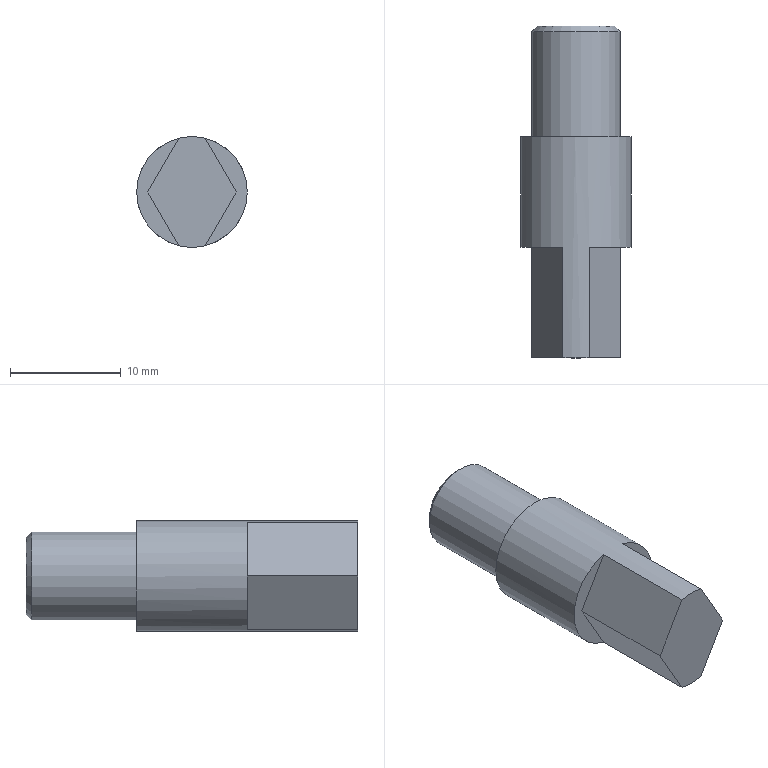Component | NX | DIAMOND_LOCATING_PIN | 1 solid | 12 faces | box 10 x 30 x 10 mm | volume 1794 mm3 | plane 9 | cylinder 2 | cone 1 | commonest cylinder face diameters 8 x1 10 x1
STEP:
#1=CARTESIAN_POINT('',(0.,0.,0.));
#2=DIRECTION('',(0.,0.,1.));
#3=DIRECTION('',(1.,0.,0.));
#4=AXIS2_PLACEMENT_3D('',#1,#2,#3);
#5=CARTESIAN_POINT('',(36.,60.,-189.));
#6=VERTEX_POINT('',#5);
#7=CARTESIAN_POINT('',(38.803,60.,-193.855));
#8=VERTEX_POINT('',#7);
#9=CARTESIAN_POINT('',(36.,60.,-189.));
#10=DIRECTION('',(0.5,0.,-0.866));
#11=VECTOR('',#10,1.);
#12=LINE('',#9,#11);
#13=CARTESIAN_POINT('',(40.,60.,-189.));
#14=DIRECTION('',(0.,-1.,0.));
#15=DIRECTION('',(1.,0.,0.));
#16=AXIS2_PLACEMENT_3D('',#13,#14,#15);
#17=PLANE('',#16);
#18=CARTESIAN_POINT('',(-4.,0.));
#19=DIRECTION('',(0.5,-0.866));
#20=VECTOR('',#19,1.);
#21=LINE('',#18,#20);
#22=(GEOMETRIC_REPRESENTATION_CONTEXT(2)PARAMETRIC_REPRESENTATION_CONTEXT()REPRESENTATION_CONTEXT('',''));
#23=DEFINITIONAL_REPRESENTATION('',(#21),#22);
#24=PCURVE('',#17,#23);
#25=CARTESIAN_POINT('',(36.,50.,-189.));
#26=DIRECTION('',(0.866,0.,0.5));
#27=DIRECTION('',(-0.5,0.,0.866));
#28=AXIS2_PLACEMENT_3D('',#25,#26,#27);
#29=PLANE('',#28);
#30=CARTESIAN_POINT('',(0.,-10.));
#31=DIRECTION('',(-1.,0.));
#32=VECTOR('',#31,1.);
#33=LINE('',#30,#32);
#34=(GEOMETRIC_REPRESENTATION_CONTEXT(2)PARAMETRIC_REPRESENTATION_CONTEXT()REPRESENTATION_CONTEXT('',''));
#35=DEFINITIONAL_REPRESENTATION('',(#33),#34);
#36=PCURVE('',#29,#35);
#37=SURFACE_CURVE('',#12,(#24,#36),.PCURVE_S1.);
#38=EDGE_CURVE('',#6,#8,#37,.T.);
#39=ORIENTED_EDGE('',*,*,#38,.F.);
#40=CARTESIAN_POINT('',(38.803,60.,-184.145));
#41=VERTEX_POINT('',#40);
#42=CARTESIAN_POINT('',(38.803,60.,-184.145));
#43=DIRECTION('',(-0.5,0.,-0.866));
#44=VECTOR('',#43,1.);
#45=LINE('',#42,#44);
#46=CARTESIAN_POINT('',(-1.197,4.855));
#47=DIRECTION('',(-0.5,-0.866));
#48=VECTOR('',#47,1.);
#49=LINE('',#46,#48);
#50=(GEOMETRIC_REPRESENTATION_CONTEXT(2)PARAMETRIC_REPRESENTATION_CONTEXT()REPRESENTATION_CONTEXT('',''));
#51=DEFINITIONAL_REPRESENTATION('',(#49),#50);
#52=PCURVE('',#17,#51);
#53=CARTESIAN_POINT('',(38.803,50.,-184.145));
#54=DIRECTION('',(0.866,0.,-0.5));
#55=DIRECTION('',(0.5,0.,0.866));
#56=AXIS2_PLACEMENT_3D('',#53,#54,#55);
#57=PLANE('',#56);
#58=CARTESIAN_POINT('',(0.,-10.));
#59=DIRECTION('',(-1.,0.));
#60=VECTOR('',#59,1.);
#61=LINE('',#58,#60);
#62=(GEOMETRIC_REPRESENTATION_CONTEXT(2)PARAMETRIC_REPRESENTATION_CONTEXT()REPRESENTATION_CONTEXT('',''));
#63=DEFINITIONAL_REPRESENTATION('',(#61),#62);
#64=PCURVE('',#57,#63);
#65=SURFACE_CURVE('',#45,(#52,#64),.PCURVE_S1.);
#66=EDGE_CURVE('',#41,#6,#65,.T.);
#67=ORIENTED_EDGE('',*,*,#66,.F.);
#68=CARTESIAN_POINT('',(40.,60.,-189.));
#69=DIRECTION('',(0.,-1.,0.));
#70=DIRECTION('',(1.,0.,0.));
#71=AXIS2_PLACEMENT_3D('',#68,#69,#70);
#72=CIRCLE('',#71,5.);
#73=CARTESIAN_POINT('',(0.,0.));
#74=DIRECTION('',(1.,0.));
#75=AXIS2_PLACEMENT_2D('',#73,#74);
#76=CIRCLE('',#75,5.);
#77=(GEOMETRIC_REPRESENTATION_CONTEXT(2)PARAMETRIC_REPRESENTATION_CONTEXT()REPRESENTATION_CONTEXT('',''));
#78=DEFINITIONAL_REPRESENTATION('',(#76),#77);
#79=PCURVE('',#17,#78);
#80=CARTESIAN_POINT('',(40.,60.,-189.));
#81=DIRECTION('',(0.,1.,0.));
#82=DIRECTION('',(-1.,0.,0.));
#83=AXIS2_PLACEMENT_3D('',#80,#81,#82);
#84=CYLINDRICAL_SURFACE('',#83,5.);
#85=CARTESIAN_POINT('',(9.425,0.));
#86=DIRECTION('',(-1.,0.));
#87=VECTOR('',#86,1.);
#88=LINE('',#85,#87);
#89=(GEOMETRIC_REPRESENTATION_CONTEXT(2)PARAMETRIC_REPRESENTATION_CONTEXT()REPRESENTATION_CONTEXT('',''));
#90=DEFINITIONAL_REPRESENTATION('',(#88),#89);
#91=PCURVE('',#84,#90);
#92=SURFACE_CURVE('',#72,(#79,#91),.PCURVE_S1.);
#93=EDGE_CURVE('',#41,#8,#92,.T.);
#94=ORIENTED_EDGE('',*,*,#93,.T.);
#95=EDGE_LOOP('',(#39,#67,#94));
#96=FACE_BOUND('',#95,.T.);
#97=ADVANCED_FACE('',(#96),#17,.T.);
#98=CARTESIAN_POINT('',(44.,79.5,-189.));
#99=VERTEX_POINT('',#98);
#100=CARTESIAN_POINT('',(40.,79.5,-189.));
#101=DIRECTION('',(0.,-1.,0.));
#102=DIRECTION('',(1.,0.,0.));
#103=AXIS2_PLACEMENT_3D('',#100,#101,#102);
#104=CIRCLE('',#103,4.);
#105=CARTESIAN_POINT('',(40.,70.,-189.));
#106=DIRECTION('',(0.,1.,0.));
#107=DIRECTION('',(-1.,0.,0.));
#108=AXIS2_PLACEMENT_3D('',#105,#106,#107);
#109=CYLINDRICAL_SURFACE('',#108,4.);
#110=CARTESIAN_POINT('',(9.425,9.5));
#111=DIRECTION('',(-1.,0.));
#112=VECTOR('',#111,1.);
#113=LINE('',#110,#112);
#114=(GEOMETRIC_REPRESENTATION_CONTEXT(2)PARAMETRIC_REPRESENTATION_CONTEXT()REPRESENTATION_CONTEXT('',''));
#115=DEFINITIONAL_REPRESENTATION('',(#113),#114);
#116=PCURVE('',#109,#115);
#117=CARTESIAN_POINT('',(40.,79.5,-189.));
#118=DIRECTION('',(0.,-1.,0.));
#119=DIRECTION('',(1.,0.,0.));
#120=AXIS2_PLACEMENT_3D('',#117,#118,#119);
#121=CONICAL_SURFACE('',#120,4.,0.7854);
#122=CARTESIAN_POINT('',(0.,0.));
#123=DIRECTION('',(1.,0.));
#124=VECTOR('',#123,1.);
#125=LINE('',#122,#124);
#126=(GEOMETRIC_REPRESENTATION_CONTEXT(2)PARAMETRIC_REPRESENTATION_CONTEXT()REPRESENTATION_CONTEXT('',''));
#127=DEFINITIONAL_REPRESENTATION('',(#125),#126);
#128=PCURVE('',#121,#127);
#129=SURFACE_CURVE('',#104,(#116,#128),.PCURVE_S1.);
#130=EDGE_CURVE('',#99,#99,#129,.T.);
#131=ORIENTED_EDGE('',*,*,#130,.T.);
#132=CARTESIAN_POINT('',(44.,70.,-189.));
#133=VERTEX_POINT('',#132);
#134=CARTESIAN_POINT('',(44.,70.,-189.));
#135=CARTESIAN_POINT('',(44.,79.5,-189.));
#136=B_SPLINE_CURVE_WITH_KNOTS('',1,(#134,#135),.UNSPECIFIED.,.F.,.F.,(2,2),(0.,9.5),.PIECEWISE_BEZIER_KNOTS.);
#137=CARTESIAN_POINT('',(3.142,0.));
#138=DIRECTION('',(0.,1.));
#139=VECTOR('',#138,1.);
#140=LINE('',#137,#139);
#141=(GEOMETRIC_REPRESENTATION_CONTEXT(2)PARAMETRIC_REPRESENTATION_CONTEXT()REPRESENTATION_CONTEXT('',''));
#142=DEFINITIONAL_REPRESENTATION('',(#140),#141);
#143=PCURVE('',#109,#142);
#144=CARTESIAN_POINT('',(9.425,0.));
#145=DIRECTION('',(0.,1.));
#146=VECTOR('',#145,1.);
#147=LINE('',#144,#146);
#148=(GEOMETRIC_REPRESENTATION_CONTEXT(2)PARAMETRIC_REPRESENTATION_CONTEXT()REPRESENTATION_CONTEXT('',''));
#149=DEFINITIONAL_REPRESENTATION('',(#147),#148);
#150=PCURVE('',#109,#149);
#151=SEAM_CURVE('',#136,(#143,#150),.PCURVE_S1.);
#152=EDGE_CURVE('',#133,#99,#151,.T.);
#153=ORIENTED_EDGE('',*,*,#152,.F.);
#154=CARTESIAN_POINT('',(40.,70.,-189.));
#155=DIRECTION('',(0.,-1.,0.));
#156=DIRECTION('',(1.,0.,0.));
#157=AXIS2_PLACEMENT_3D('',#154,#155,#156);
#158=CIRCLE('',#157,4.);
#159=CARTESIAN_POINT('',(9.425,0.));
#160=DIRECTION('',(-1.,0.));
#161=VECTOR('',#160,1.);
#162=LINE('',#159,#161);
#163=(GEOMETRIC_REPRESENTATION_CONTEXT(2)PARAMETRIC_REPRESENTATION_CONTEXT()REPRESENTATION_CONTEXT('',''));
#164=DEFINITIONAL_REPRESENTATION('',(#162),#163);
#165=PCURVE('',#109,#164);
#166=CARTESIAN_POINT('',(40.,70.,-189.));
#167=DIRECTION('',(0.,-1.,0.));
#168=DIRECTION('',(1.,0.,0.));
#169=AXIS2_PLACEMENT_3D('',#166,#167,#168);
#170=PLANE('',#169);
#171=CARTESIAN_POINT('',(0.,0.));
#172=DIRECTION('',(1.,0.));
#173=AXIS2_PLACEMENT_2D('',#171,#172);
#174=CIRCLE('',#173,4.);
#175=(GEOMETRIC_REPRESENTATION_CONTEXT(2)PARAMETRIC_REPRESENTATION_CONTEXT()REPRESENTATION_CONTEXT('',''));
#176=DEFINITIONAL_REPRESENTATION('',(#174),#175);
#177=PCURVE('',#170,#176);
#178=SURFACE_CURVE('',#158,(#165,#177),.PCURVE_S1.);
#179=EDGE_CURVE('',#133,#133,#178,.T.);
#180=ORIENTED_EDGE('',*,*,#179,.F.);
#181=ORIENTED_EDGE('',*,*,#152,.T.);
#182=EDGE_LOOP('',(#131,#153,#180,#181));
#183=FACE_BOUND('',#182,.T.);
#184=ADVANCED_FACE('',(#183),#109,.T.);
#185=CARTESIAN_POINT('',(43.5,80.,-189.));
#186=VERTEX_POINT('',#185);
#187=CARTESIAN_POINT('',(40.,80.,-189.));
#188=DIRECTION('',(0.,1.,0.));
#189=DIRECTION('',(1.,0.,0.));
#190=AXIS2_PLACEMENT_3D('',#187,#188,#189);
#191=CIRCLE('',#190,3.5);
#192=CARTESIAN_POINT('',(40.,80.,-189.));
#193=DIRECTION('',(0.,-1.,0.));
#194=DIRECTION('',(1.,0.,0.));
#195=AXIS2_PLACEMENT_3D('',#192,#193,#194);
#196=PLANE('',#195);
#197=CARTESIAN_POINT('',(3.5,0.));
#198=CARTESIAN_POINT('',(3.5,-6.062));
#199=CARTESIAN_POINT('',(-1.75,-3.031));
#200=CARTESIAN_POINT('',(-7.,-0.));
#201=CARTESIAN_POINT('',(-1.75,3.031));
#202=CARTESIAN_POINT('',(3.5,6.062));
#203=CARTESIAN_POINT('',(3.5,0.));
#204=(BOUNDED_CURVE()B_SPLINE_CURVE(2,(#197,#198,#199,#200,#201,#202,#203),.UNSPECIFIED.,.T.,.F.)B_SPLINE_CURVE_WITH_KNOTS((1,2,2,2,2,1),(-2.094,0.,2.094,4.189,6.283,8.378),.UNSPECIFIED.)CURVE()GEOMETRIC_REPRESENTATION_ITEM()RATIONAL_B_SPLINE_CURVE((1.,0.5,1.,0.5,1.,0.5,1.))REPRESENTATION_ITEM(''));
#205=(GEOMETRIC_REPRESENTATION_CONTEXT(2)PARAMETRIC_REPRESENTATION_CONTEXT()REPRESENTATION_CONTEXT('',''));
#206=DEFINITIONAL_REPRESENTATION('',(#204),#205);
#207=PCURVE('',#196,#206);
#208=CARTESIAN_POINT('',(6.283,-0.5));
#209=DIRECTION('',(-1.,0.));
#210=VECTOR('',#209,1.);
#211=LINE('',#208,#210);
#212=(GEOMETRIC_REPRESENTATION_CONTEXT(2)PARAMETRIC_REPRESENTATION_CONTEXT()REPRESENTATION_CONTEXT('',''));
#213=DEFINITIONAL_REPRESENTATION('',(#211),#212);
#214=PCURVE('',#121,#213);
#215=SURFACE_CURVE('',#191,(#207,#214),.PCURVE_S1.);
#216=EDGE_CURVE('',#186,#186,#215,.T.);
#217=ORIENTED_EDGE('',*,*,#216,.T.);
#218=EDGE_LOOP('',(#217));
#219=FACE_BOUND('',#218,.T.);
#220=ADVANCED_FACE('',(#219),#196,.F.);
#221=ORIENTED_EDGE('',*,*,#93,.F.);
#222=CARTESIAN_POINT('',(38.803,70.,-184.145));
#223=VERTEX_POINT('',#222);
#224=CARTESIAN_POINT('',(38.803,60.,-184.145));
#225=CARTESIAN_POINT('',(38.803,70.,-184.145));
#226=B_SPLINE_CURVE_WITH_KNOTS('',1,(#224,#225),.UNSPECIFIED.,.F.,.F.,(2,2),(0.,10.),.PIECEWISE_BEZIER_KNOTS.);
#227=CARTESIAN_POINT('',(7.612,0.));
#228=DIRECTION('',(0.,1.));
#229=VECTOR('',#228,1.);
#230=LINE('',#227,#229);
#231=(GEOMETRIC_REPRESENTATION_CONTEXT(2)PARAMETRIC_REPRESENTATION_CONTEXT()REPRESENTATION_CONTEXT('',''));
#232=DEFINITIONAL_REPRESENTATION('',(#230),#231);
#233=PCURVE('',#84,#232);
#234=CARTESIAN_POINT('',(1.329,0.));
#235=DIRECTION('',(0.,1.));
#236=VECTOR('',#235,1.);
#237=LINE('',#234,#236);
#238=(GEOMETRIC_REPRESENTATION_CONTEXT(2)PARAMETRIC_REPRESENTATION_CONTEXT()REPRESENTATION_CONTEXT('',''));
#239=DEFINITIONAL_REPRESENTATION('',(#237),#238);
#240=PCURVE('',#84,#239);
#241=SEAM_CURVE('',#226,(#233,#240),.PCURVE_S1.);
#242=EDGE_CURVE('',#41,#223,#241,.T.);
#243=ORIENTED_EDGE('',*,*,#242,.T.);
#244=CARTESIAN_POINT('',(45.,70.,-189.));
#245=VERTEX_POINT('',#244);
#246=CARTESIAN_POINT('',(40.,70.,-189.));
#247=DIRECTION('',(0.,-1.,0.));
#248=DIRECTION('',(1.,0.,0.));
#249=AXIS2_PLACEMENT_3D('',#246,#247,#248);
#250=CIRCLE('',#249,5.);
#251=CARTESIAN_POINT('',(9.425,10.));
#252=DIRECTION('',(-1.,0.));
#253=VECTOR('',#252,1.);
#254=LINE('',#251,#253);
#255=(GEOMETRIC_REPRESENTATION_CONTEXT(2)PARAMETRIC_REPRESENTATION_CONTEXT()REPRESENTATION_CONTEXT('',''));
#256=DEFINITIONAL_REPRESENTATION('',(#254),#255);
#257=PCURVE('',#84,#256);
#258=CARTESIAN_POINT('',(0.,0.));
#259=DIRECTION('',(1.,0.));
#260=AXIS2_PLACEMENT_2D('',#258,#259);
#261=CIRCLE('',#260,5.);
#262=(GEOMETRIC_REPRESENTATION_CONTEXT(2)PARAMETRIC_REPRESENTATION_CONTEXT()REPRESENTATION_CONTEXT('',''));
#263=DEFINITIONAL_REPRESENTATION('',(#261),#262);
#264=PCURVE('',#170,#263);
#265=SURFACE_CURVE('',#250,(#257,#264),.PCURVE_S1.);
#266=EDGE_CURVE('',#223,#245,#265,.T.);
#267=ORIENTED_EDGE('',*,*,#266,.T.);
#268=CARTESIAN_POINT('',(40.,70.,-189.));
#269=DIRECTION('',(0.,-1.,0.));
#270=DIRECTION('',(1.,0.,0.));
#271=AXIS2_PLACEMENT_3D('',#268,#269,#270);
#272=CIRCLE('',#271,5.);
#273=CARTESIAN_POINT('',(3.142,10.));
#274=DIRECTION('',(-1.,0.));
#275=VECTOR('',#274,1.);
#276=LINE('',#273,#275);
#277=(GEOMETRIC_REPRESENTATION_CONTEXT(2)PARAMETRIC_REPRESENTATION_CONTEXT()REPRESENTATION_CONTEXT('',''));
#278=DEFINITIONAL_REPRESENTATION('',(#276),#277);
#279=PCURVE('',#84,#278);
#280=CARTESIAN_POINT('',(0.,0.));
#281=DIRECTION('',(1.,0.));
#282=AXIS2_PLACEMENT_2D('',#280,#281);
#283=CIRCLE('',#282,5.);
#284=(GEOMETRIC_REPRESENTATION_CONTEXT(2)PARAMETRIC_REPRESENTATION_CONTEXT()REPRESENTATION_CONTEXT('',''));
#285=DEFINITIONAL_REPRESENTATION('',(#283),#284);
#286=PCURVE('',#170,#285);
#287=SURFACE_CURVE('',#272,(#279,#286),.PCURVE_S1.);
#288=EDGE_CURVE('',#245,#223,#287,.T.);
#289=ORIENTED_EDGE('',*,*,#288,.T.);
#290=ORIENTED_EDGE('',*,*,#242,.F.);
#291=CARTESIAN_POINT('',(38.803,50.,-184.145));
#292=VERTEX_POINT('',#291);
#293=CARTESIAN_POINT('',(38.803,50.,-184.145));
#294=DIRECTION('',(0.,1.,0.));
#295=VECTOR('',#294,1.);
#296=LINE('',#293,#295);
#297=CARTESIAN_POINT('',(1.329,-10.));
#298=DIRECTION('',(0.,1.));
#299=VECTOR('',#298,1.);
#300=LINE('',#297,#299);
#301=(GEOMETRIC_REPRESENTATION_CONTEXT(2)PARAMETRIC_REPRESENTATION_CONTEXT()REPRESENTATION_CONTEXT('',''));
#302=DEFINITIONAL_REPRESENTATION('',(#300),#301);
#303=PCURVE('',#84,#302);
#304=CARTESIAN_POINT('',(0.,0.));
#305=DIRECTION('',(0.,-1.));
#306=VECTOR('',#305,1.);
#307=LINE('',#304,#306);
#308=(GEOMETRIC_REPRESENTATION_CONTEXT(2)PARAMETRIC_REPRESENTATION_CONTEXT()REPRESENTATION_CONTEXT('',''));
#309=DEFINITIONAL_REPRESENTATION('',(#307),#308);
#310=PCURVE('',#57,#309);
#311=SURFACE_CURVE('',#296,(#303,#310),.PCURVE_S1.);
#312=EDGE_CURVE('',#292,#41,#311,.T.);
#313=ORIENTED_EDGE('',*,*,#312,.F.);
#314=CARTESIAN_POINT('',(41.197,50.,-184.145));
#315=VERTEX_POINT('',#314);
#316=CARTESIAN_POINT('',(40.,50.,-189.));
#317=DIRECTION('',(0.,-1.,0.));
#318=DIRECTION('',(1.,0.,0.));
#319=AXIS2_PLACEMENT_3D('',#316,#317,#318);
#320=CIRCLE('',#319,5.);
#321=CARTESIAN_POINT('',(3.142,-10.));
#322=DIRECTION('',(-1.,0.));
#323=VECTOR('',#322,1.);
#324=LINE('',#321,#323);
#325=(GEOMETRIC_REPRESENTATION_CONTEXT(2)PARAMETRIC_REPRESENTATION_CONTEXT()REPRESENTATION_CONTEXT('',''));
#326=DEFINITIONAL_REPRESENTATION('',(#324),#325);
#327=PCURVE('',#84,#326);
#328=CARTESIAN_POINT('',(40.,50.,-189.));
#329=DIRECTION('',(0.,-1.,0.));
#330=DIRECTION('',(1.,0.,0.));
#331=AXIS2_PLACEMENT_3D('',#328,#329,#330);
#332=PLANE('',#331);
#333=CARTESIAN_POINT('',(0.,0.));
#334=DIRECTION('',(1.,0.));
#335=AXIS2_PLACEMENT_2D('',#333,#334);
#336=CIRCLE('',#335,5.);
#337=(GEOMETRIC_REPRESENTATION_CONTEXT(2)PARAMETRIC_REPRESENTATION_CONTEXT()REPRESENTATION_CONTEXT('',''));
#338=DEFINITIONAL_REPRESENTATION('',(#336),#337);
#339=PCURVE('',#332,#338);
#340=SURFACE_CURVE('',#320,(#327,#339),.PCURVE_S1.);
#341=EDGE_CURVE('',#315,#292,#340,.T.);
#342=ORIENTED_EDGE('',*,*,#341,.F.);
#343=CARTESIAN_POINT('',(41.197,60.,-184.145));
#344=VERTEX_POINT('',#343);
#345=CARTESIAN_POINT('',(41.197,50.,-184.145));
#346=DIRECTION('',(0.,1.,0.));
#347=VECTOR('',#346,1.);
#348=LINE('',#345,#347);
#349=CARTESIAN_POINT('',(1.813,-10.));
#350=DIRECTION('',(0.,1.));
#351=VECTOR('',#350,1.);
#352=LINE('',#349,#351);
#353=(GEOMETRIC_REPRESENTATION_CONTEXT(2)PARAMETRIC_REPRESENTATION_CONTEXT()REPRESENTATION_CONTEXT('',''));
#354=DEFINITIONAL_REPRESENTATION('',(#352),#353);
#355=PCURVE('',#84,#354);
#356=CARTESIAN_POINT('',(44.,50.,-189.));
#357=DIRECTION('',(-0.866,0.,-0.5));
#358=DIRECTION('',(0.5,0.,-0.866));
#359=AXIS2_PLACEMENT_3D('',#356,#357,#358);
#360=PLANE('',#359);
#361=CARTESIAN_POINT('',(-5.606,0.));
#362=DIRECTION('',(0.,-1.));
#363=VECTOR('',#362,1.);
#364=LINE('',#361,#363);
#365=(GEOMETRIC_REPRESENTATION_CONTEXT(2)PARAMETRIC_REPRESENTATION_CONTEXT()REPRESENTATION_CONTEXT('',''));
#366=DEFINITIONAL_REPRESENTATION('',(#364),#365);
#367=PCURVE('',#360,#366);
#368=SURFACE_CURVE('',#348,(#355,#367),.PCURVE_S1.);
#369=EDGE_CURVE('',#315,#344,#368,.T.);
#370=ORIENTED_EDGE('',*,*,#369,.T.);
#371=CARTESIAN_POINT('',(41.197,60.,-193.855));
#372=VERTEX_POINT('',#371);
#373=CARTESIAN_POINT('',(40.,60.,-189.));
#374=DIRECTION('',(0.,-1.,0.));
#375=DIRECTION('',(1.,0.,0.));
#376=AXIS2_PLACEMENT_3D('',#373,#374,#375);
#377=CIRCLE('',#376,5.);
#378=CARTESIAN_POINT('',(9.425,0.));
#379=DIRECTION('',(-1.,0.));
#380=VECTOR('',#379,1.);
#381=LINE('',#378,#380);
#382=(GEOMETRIC_REPRESENTATION_CONTEXT(2)PARAMETRIC_REPRESENTATION_CONTEXT()REPRESENTATION_CONTEXT('',''));
#383=DEFINITIONAL_REPRESENTATION('',(#381),#382);
#384=PCURVE('',#84,#383);
#385=CARTESIAN_POINT('',(40.,60.,-189.));
#386=DIRECTION('',(0.,-1.,0.));
#387=DIRECTION('',(1.,0.,0.));
#388=AXIS2_PLACEMENT_3D('',#385,#386,#387);
#389=PLANE('',#388);
#390=CARTESIAN_POINT('',(0.,0.));
#391=DIRECTION('',(1.,0.));
#392=AXIS2_PLACEMENT_2D('',#390,#391);
#393=CIRCLE('',#392,5.);
#394=(GEOMETRIC_REPRESENTATION_CONTEXT(2)PARAMETRIC_REPRESENTATION_CONTEXT()REPRESENTATION_CONTEXT('',''));
#395=DEFINITIONAL_REPRESENTATION('',(#393),#394);
#396=PCURVE('',#389,#395);
#397=SURFACE_CURVE('',#377,(#384,#396),.PCURVE_S1.);
#398=EDGE_CURVE('',#372,#344,#397,.T.);
#399=ORIENTED_EDGE('',*,*,#398,.F.);
#400=CARTESIAN_POINT('',(41.197,50.,-193.855));
#401=VERTEX_POINT('',#400);
#402=CARTESIAN_POINT('',(41.197,50.,-193.855));
#403=DIRECTION('',(0.,1.,0.));
#404=VECTOR('',#403,1.);
#405=LINE('',#402,#404);
#406=CARTESIAN_POINT('',(4.471,-10.));
#407=DIRECTION('',(0.,1.));
#408=VECTOR('',#407,1.);
#409=LINE('',#406,#408);
#410=(GEOMETRIC_REPRESENTATION_CONTEXT(2)PARAMETRIC_REPRESENTATION_CONTEXT()REPRESENTATION_CONTEXT('',''));
#411=DEFINITIONAL_REPRESENTATION('',(#409),#410);
#412=PCURVE('',#84,#411);
#413=CARTESIAN_POINT('',(41.197,50.,-193.855));
#414=DIRECTION('',(-0.866,0.,0.5));
#415=DIRECTION('',(-0.5,0.,-0.866));
#416=AXIS2_PLACEMENT_3D('',#413,#414,#415);
#417=PLANE('',#416);
#418=CARTESIAN_POINT('',(-0.,0.));
#419=DIRECTION('',(0.,-1.));
#420=VECTOR('',#419,1.);
#421=LINE('',#418,#420);
#422=(GEOMETRIC_REPRESENTATION_CONTEXT(2)PARAMETRIC_REPRESENTATION_CONTEXT()REPRESENTATION_CONTEXT('',''));
#423=DEFINITIONAL_REPRESENTATION('',(#421),#422);
#424=PCURVE('',#417,#423);
#425=SURFACE_CURVE('',#405,(#412,#424),.PCURVE_S1.);
#426=EDGE_CURVE('',#401,#372,#425,.T.);
#427=ORIENTED_EDGE('',*,*,#426,.F.);
#428=CARTESIAN_POINT('',(38.803,50.,-193.855));
#429=VERTEX_POINT('',#428);
#430=CARTESIAN_POINT('',(40.,50.,-189.));
#431=DIRECTION('',(0.,-1.,0.));
#432=DIRECTION('',(1.,0.,0.));
#433=AXIS2_PLACEMENT_3D('',#430,#431,#432);
#434=CIRCLE('',#433,5.);
#435=CARTESIAN_POINT('',(9.425,-10.));
#436=DIRECTION('',(-1.,0.));
#437=VECTOR('',#436,1.);
#438=LINE('',#435,#437);
#439=(GEOMETRIC_REPRESENTATION_CONTEXT(2)PARAMETRIC_REPRESENTATION_CONTEXT()REPRESENTATION_CONTEXT('',''));
#440=DEFINITIONAL_REPRESENTATION('',(#438),#439);
#441=PCURVE('',#84,#440);
#442=CARTESIAN_POINT('',(0.,0.));
#443=DIRECTION('',(1.,0.));
#444=AXIS2_PLACEMENT_2D('',#442,#443);
#445=CIRCLE('',#444,5.);
#446=(GEOMETRIC_REPRESENTATION_CONTEXT(2)PARAMETRIC_REPRESENTATION_CONTEXT()REPRESENTATION_CONTEXT('',''));
#447=DEFINITIONAL_REPRESENTATION('',(#445),#446);
#448=PCURVE('',#332,#447);
#449=SURFACE_CURVE('',#434,(#441,#448),.PCURVE_S1.);
#450=EDGE_CURVE('',#429,#401,#449,.T.);
#451=ORIENTED_EDGE('',*,*,#450,.F.);
#452=CARTESIAN_POINT('',(38.803,50.,-193.855));
#453=DIRECTION('',(0.,1.,0.));
#454=VECTOR('',#453,1.);
#455=LINE('',#452,#454);
#456=CARTESIAN_POINT('',(4.954,-10.));
#457=DIRECTION('',(0.,1.));
#458=VECTOR('',#457,1.);
#459=LINE('',#456,#458);
#460=(GEOMETRIC_REPRESENTATION_CONTEXT(2)PARAMETRIC_REPRESENTATION_CONTEXT()REPRESENTATION_CONTEXT('',''));
#461=DEFINITIONAL_REPRESENTATION('',(#459),#460);
#462=PCURVE('',#84,#461);
#463=CARTESIAN_POINT('',(-5.606,0.));
#464=DIRECTION('',(0.,-1.));
#465=VECTOR('',#464,1.);
#466=LINE('',#463,#465);
#467=(GEOMETRIC_REPRESENTATION_CONTEXT(2)PARAMETRIC_REPRESENTATION_CONTEXT()REPRESENTATION_CONTEXT('',''));
#468=DEFINITIONAL_REPRESENTATION('',(#466),#467);
#469=PCURVE('',#29,#468);
#470=SURFACE_CURVE('',#455,(#462,#469),.PCURVE_S1.);
#471=EDGE_CURVE('',#429,#8,#470,.T.);
#472=ORIENTED_EDGE('',*,*,#471,.T.);
#473=EDGE_LOOP('',(#221,#243,#267,#289,#290,#313,#342,#370,#399,#427,#451,#472));
#474=FACE_BOUND('',#473,.T.);
#475=ADVANCED_FACE('',(#474),#84,.T.);
#476=CARTESIAN_POINT('',(44.,60.,-189.));
#477=VERTEX_POINT('',#476);
#478=CARTESIAN_POINT('',(44.,60.,-189.));
#479=DIRECTION('',(-0.5,0.,0.866));
#480=VECTOR('',#479,1.);
#481=LINE('',#478,#480);
#482=CARTESIAN_POINT('',(4.,0.));
#483=DIRECTION('',(-0.5,0.866));
#484=VECTOR('',#483,1.);
#485=LINE('',#482,#484);
#486=(GEOMETRIC_REPRESENTATION_CONTEXT(2)PARAMETRIC_REPRESENTATION_CONTEXT()REPRESENTATION_CONTEXT('',''));
#487=DEFINITIONAL_REPRESENTATION('',(#485),#486);
#488=PCURVE('',#389,#487);
#489=CARTESIAN_POINT('',(0.,-10.));
#490=DIRECTION('',(-1.,0.));
#491=VECTOR('',#490,1.);
#492=LINE('',#489,#491);
#493=(GEOMETRIC_REPRESENTATION_CONTEXT(2)PARAMETRIC_REPRESENTATION_CONTEXT()REPRESENTATION_CONTEXT('',''));
#494=DEFINITIONAL_REPRESENTATION('',(#492),#493);
#495=PCURVE('',#360,#494);
#496=SURFACE_CURVE('',#481,(#488,#495),.PCURVE_S1.);
#497=EDGE_CURVE('',#477,#344,#496,.T.);
#498=ORIENTED_EDGE('',*,*,#497,.F.);
#499=CARTESIAN_POINT('',(41.197,60.,-193.855));
#500=DIRECTION('',(0.5,0.,0.866));
#501=VECTOR('',#500,1.);
#502=LINE('',#499,#501);
#503=CARTESIAN_POINT('',(1.197,-4.855));
#504=DIRECTION('',(0.5,0.866));
#505=VECTOR('',#504,1.);
#506=LINE('',#503,#505);
#507=(GEOMETRIC_REPRESENTATION_CONTEXT(2)PARAMETRIC_REPRESENTATION_CONTEXT()REPRESENTATION_CONTEXT('',''));
#508=DEFINITIONAL_REPRESENTATION('',(#506),#507);
#509=PCURVE('',#389,#508);
#510=CARTESIAN_POINT('',(0.,-10.));
#511=DIRECTION('',(-1.,0.));
#512=VECTOR('',#511,1.);
#513=LINE('',#510,#512);
#514=(GEOMETRIC_REPRESENTATION_CONTEXT(2)PARAMETRIC_REPRESENTATION_CONTEXT()REPRESENTATION_CONTEXT('',''));
#515=DEFINITIONAL_REPRESENTATION('',(#513),#514);
#516=PCURVE('',#417,#515);
#517=SURFACE_CURVE('',#502,(#509,#516),.PCURVE_S1.);
#518=EDGE_CURVE('',#372,#477,#517,.T.);
#519=ORIENTED_EDGE('',*,*,#518,.F.);
#520=ORIENTED_EDGE('',*,*,#398,.T.);
#521=EDGE_LOOP('',(#498,#519,#520));
#522=FACE_BOUND('',#521,.T.);
#523=ADVANCED_FACE('',(#522),#389,.T.);
#524=ORIENTED_EDGE('',*,*,#179,.T.);
#525=EDGE_LOOP('',(#524));
#526=FACE_BOUND('',#525,.T.);
#527=ORIENTED_EDGE('',*,*,#288,.F.);
#528=ORIENTED_EDGE('',*,*,#266,.F.);
#529=EDGE_LOOP('',(#527,#528));
#530=FACE_BOUND('',#529,.T.);
#531=ADVANCED_FACE('',(#526,#530),#170,.F.);
#532=ORIENTED_EDGE('',*,*,#38,.T.);
#533=ORIENTED_EDGE('',*,*,#471,.F.);
#534=CARTESIAN_POINT('',(36.,50.,-189.));
#535=VERTEX_POINT('',#534);
#536=CARTESIAN_POINT('',(36.,50.,-189.));
#537=DIRECTION('',(0.5,0.,-0.866));
#538=VECTOR('',#537,1.);
#539=LINE('',#536,#538);
#540=CARTESIAN_POINT('',(0.,0.));
#541=DIRECTION('',(-1.,0.));
#542=VECTOR('',#541,1.);
#543=LINE('',#540,#542);
#544=(GEOMETRIC_REPRESENTATION_CONTEXT(2)PARAMETRIC_REPRESENTATION_CONTEXT()REPRESENTATION_CONTEXT('',''));
#545=DEFINITIONAL_REPRESENTATION('',(#543),#544);
#546=PCURVE('',#29,#545);
#547=CARTESIAN_POINT('',(-4.,0.));
#548=DIRECTION('',(0.5,-0.866));
#549=VECTOR('',#548,1.);
#550=LINE('',#547,#549);
#551=(GEOMETRIC_REPRESENTATION_CONTEXT(2)PARAMETRIC_REPRESENTATION_CONTEXT()REPRESENTATION_CONTEXT('',''));
#552=DEFINITIONAL_REPRESENTATION('',(#550),#551);
#553=PCURVE('',#332,#552);
#554=SURFACE_CURVE('',#539,(#546,#553),.PCURVE_S1.);
#555=EDGE_CURVE('',#535,#429,#554,.T.);
#556=ORIENTED_EDGE('',*,*,#555,.F.);
#557=CARTESIAN_POINT('',(36.,50.,-189.));
#558=DIRECTION('',(0.,1.,0.));
#559=VECTOR('',#558,1.);
#560=LINE('',#557,#559);
#561=CARTESIAN_POINT('',(0.,0.));
#562=DIRECTION('',(0.,-1.));
#563=VECTOR('',#562,1.);
#564=LINE('',#561,#563);
#565=(GEOMETRIC_REPRESENTATION_CONTEXT(2)PARAMETRIC_REPRESENTATION_CONTEXT()REPRESENTATION_CONTEXT('',''));
#566=DEFINITIONAL_REPRESENTATION('',(#564),#565);
#567=PCURVE('',#29,#566);
#568=CARTESIAN_POINT('',(-5.606,0.));
#569=DIRECTION('',(0.,-1.));
#570=VECTOR('',#569,1.);
#571=LINE('',#568,#570);
#572=(GEOMETRIC_REPRESENTATION_CONTEXT(2)PARAMETRIC_REPRESENTATION_CONTEXT()REPRESENTATION_CONTEXT('',''));
#573=DEFINITIONAL_REPRESENTATION('',(#571),#572);
#574=PCURVE('',#57,#573);
#575=SURFACE_CURVE('',#560,(#567,#574),.PCURVE_S1.);
#576=EDGE_CURVE('',#535,#6,#575,.T.);
#577=ORIENTED_EDGE('',*,*,#576,.T.);
#578=EDGE_LOOP('',(#532,#533,#556,#577));
#579=FACE_BOUND('',#578,.T.);
#580=ADVANCED_FACE('',(#579),#29,.F.);
#581=ORIENTED_EDGE('',*,*,#518,.T.);
#582=CARTESIAN_POINT('',(44.,50.,-189.));
#583=VERTEX_POINT('',#582);
#584=CARTESIAN_POINT('',(44.,50.,-189.));
#585=DIRECTION('',(0.,1.,0.));
#586=VECTOR('',#585,1.);
#587=LINE('',#584,#586);
#588=CARTESIAN_POINT('',(-5.606,0.));
#589=DIRECTION('',(0.,-1.));
#590=VECTOR('',#589,1.);
#591=LINE('',#588,#590);
#592=(GEOMETRIC_REPRESENTATION_CONTEXT(2)PARAMETRIC_REPRESENTATION_CONTEXT()REPRESENTATION_CONTEXT('',''));
#593=DEFINITIONAL_REPRESENTATION('',(#591),#592);
#594=PCURVE('',#417,#593);
#595=CARTESIAN_POINT('',(0.,0.));
#596=DIRECTION('',(0.,-1.));
#597=VECTOR('',#596,1.);
#598=LINE('',#595,#597);
#599=(GEOMETRIC_REPRESENTATION_CONTEXT(2)PARAMETRIC_REPRESENTATION_CONTEXT()REPRESENTATION_CONTEXT('',''));
#600=DEFINITIONAL_REPRESENTATION('',(#598),#599);
#601=PCURVE('',#360,#600);
#602=SURFACE_CURVE('',#587,(#594,#601),.PCURVE_S1.);
#603=EDGE_CURVE('',#583,#477,#602,.T.);
#604=ORIENTED_EDGE('',*,*,#603,.F.);
#605=CARTESIAN_POINT('',(41.197,50.,-193.855));
#606=DIRECTION('',(0.5,0.,0.866));
#607=VECTOR('',#606,1.);
#608=LINE('',#605,#607);
#609=CARTESIAN_POINT('',(0.,0.));
#610=DIRECTION('',(-1.,0.));
#611=VECTOR('',#610,1.);
#612=LINE('',#609,#611);
#613=(GEOMETRIC_REPRESENTATION_CONTEXT(2)PARAMETRIC_REPRESENTATION_CONTEXT()REPRESENTATION_CONTEXT('',''));
#614=DEFINITIONAL_REPRESENTATION('',(#612),#613);
#615=PCURVE('',#417,#614);
#616=CARTESIAN_POINT('',(1.197,-4.855));
#617=DIRECTION('',(0.5,0.866));
#618=VECTOR('',#617,1.);
#619=LINE('',#616,#618);
#620=(GEOMETRIC_REPRESENTATION_CONTEXT(2)PARAMETRIC_REPRESENTATION_CONTEXT()REPRESENTATION_CONTEXT('',''));
#621=DEFINITIONAL_REPRESENTATION('',(#619),#620);
#622=PCURVE('',#332,#621);
#623=SURFACE_CURVE('',#608,(#615,#622),.PCURVE_S1.);
#624=EDGE_CURVE('',#401,#583,#623,.T.);
#625=ORIENTED_EDGE('',*,*,#624,.F.);
#626=ORIENTED_EDGE('',*,*,#426,.T.);
#627=EDGE_LOOP('',(#581,#604,#625,#626));
#628=FACE_BOUND('',#627,.T.);
#629=ADVANCED_FACE('',(#628),#417,.F.);
#630=ORIENTED_EDGE('',*,*,#497,.T.);
#631=ORIENTED_EDGE('',*,*,#369,.F.);
#632=CARTESIAN_POINT('',(44.,50.,-189.));
#633=DIRECTION('',(-0.5,0.,0.866));
#634=VECTOR('',#633,1.);
#635=LINE('',#632,#634);
#636=CARTESIAN_POINT('',(0.,0.));
#637=DIRECTION('',(-1.,0.));
#638=VECTOR('',#637,1.);
#639=LINE('',#636,#638);
#640=(GEOMETRIC_REPRESENTATION_CONTEXT(2)PARAMETRIC_REPRESENTATION_CONTEXT()REPRESENTATION_CONTEXT('',''));
#641=DEFINITIONAL_REPRESENTATION('',(#639),#640);
#642=PCURVE('',#360,#641);
#643=CARTESIAN_POINT('',(4.,0.));
#644=DIRECTION('',(-0.5,0.866));
#645=VECTOR('',#644,1.);
#646=LINE('',#643,#645);
#647=(GEOMETRIC_REPRESENTATION_CONTEXT(2)PARAMETRIC_REPRESENTATION_CONTEXT()REPRESENTATION_CONTEXT('',''));
#648=DEFINITIONAL_REPRESENTATION('',(#646),#647);
#649=PCURVE('',#332,#648);
#650=SURFACE_CURVE('',#635,(#642,#649),.PCURVE_S1.);
#651=EDGE_CURVE('',#583,#315,#650,.T.);
#652=ORIENTED_EDGE('',*,*,#651,.F.);
#653=ORIENTED_EDGE('',*,*,#603,.T.);
#654=EDGE_LOOP('',(#630,#631,#652,#653));
#655=FACE_BOUND('',#654,.T.);
#656=ADVANCED_FACE('',(#655),#360,.F.);
#657=ORIENTED_EDGE('',*,*,#66,.T.);
#658=ORIENTED_EDGE('',*,*,#576,.F.);
#659=CARTESIAN_POINT('',(38.803,50.,-184.145));
#660=DIRECTION('',(-0.5,0.,-0.866));
#661=VECTOR('',#660,1.);
#662=LINE('',#659,#661);
#663=CARTESIAN_POINT('',(0.,0.));
#664=DIRECTION('',(-1.,0.));
#665=VECTOR('',#664,1.);
#666=LINE('',#663,#665);
#667=(GEOMETRIC_REPRESENTATION_CONTEXT(2)PARAMETRIC_REPRESENTATION_CONTEXT()REPRESENTATION_CONTEXT('',''));
#668=DEFINITIONAL_REPRESENTATION('',(#666),#667);
#669=PCURVE('',#57,#668);
#670=CARTESIAN_POINT('',(-1.197,4.855));
#671=DIRECTION('',(-0.5,-0.866));
#672=VECTOR('',#671,1.);
#673=LINE('',#670,#672);
#674=(GEOMETRIC_REPRESENTATION_CONTEXT(2)PARAMETRIC_REPRESENTATION_CONTEXT()REPRESENTATION_CONTEXT('',''));
#675=DEFINITIONAL_REPRESENTATION('',(#673),#674);
#676=PCURVE('',#332,#675);
#677=SURFACE_CURVE('',#662,(#669,#676),.PCURVE_S1.);
#678=EDGE_CURVE('',#292,#535,#677,.T.);
#679=ORIENTED_EDGE('',*,*,#678,.F.);
#680=ORIENTED_EDGE('',*,*,#312,.T.);
#681=EDGE_LOOP('',(#657,#658,#679,#680));
#682=FACE_BOUND('',#681,.T.);
#683=ADVANCED_FACE('',(#682),#57,.F.);
#684=ORIENTED_EDGE('',*,*,#555,.T.);
#685=ORIENTED_EDGE('',*,*,#450,.T.);
#686=ORIENTED_EDGE('',*,*,#624,.T.);
#687=ORIENTED_EDGE('',*,*,#651,.T.);
#688=ORIENTED_EDGE('',*,*,#341,.T.);
#689=ORIENTED_EDGE('',*,*,#678,.T.);
#690=EDGE_LOOP('',(#684,#685,#686,#687,#688,#689));
#691=FACE_BOUND('',#690,.T.);
#692=ADVANCED_FACE('',(#691),#332,.T.);
#693=ORIENTED_EDGE('',*,*,#216,.F.);
#694=CARTESIAN_POINT('',(43.5,80.,-189.));
#695=CARTESIAN_POINT('',(44.,79.5,-189.));
#696=B_SPLINE_CURVE_WITH_KNOTS('',1,(#694,#695),.UNSPECIFIED.,.F.,.F.,(2,2),(-0.7071,0.),.PIECEWISE_BEZIER_KNOTS.);
#697=CARTESIAN_POINT('',(6.283,0.));
#698=DIRECTION('',(0.,1.));
#699=VECTOR('',#698,1.);
#700=LINE('',#697,#699);
#701=(GEOMETRIC_REPRESENTATION_CONTEXT(2)PARAMETRIC_REPRESENTATION_CONTEXT()REPRESENTATION_CONTEXT('',''));
#702=DEFINITIONAL_REPRESENTATION('',(#700),#701);
#703=PCURVE('',#121,#702);
#704=CARTESIAN_POINT('',(0.,0.));
#705=DIRECTION('',(0.,1.));
#706=VECTOR('',#705,1.);
#707=LINE('',#704,#706);
#708=(GEOMETRIC_REPRESENTATION_CONTEXT(2)PARAMETRIC_REPRESENTATION_CONTEXT()REPRESENTATION_CONTEXT('',''));
#709=DEFINITIONAL_REPRESENTATION('',(#707),#708);
#710=PCURVE('',#121,#709);
#711=SEAM_CURVE('',#696,(#703,#710),.PCURVE_S1.);
#712=EDGE_CURVE('',#186,#99,#711,.T.);
#713=ORIENTED_EDGE('',*,*,#712,.T.);
#714=ORIENTED_EDGE('',*,*,#130,.F.);
#715=ORIENTED_EDGE('',*,*,#712,.F.);
#716=EDGE_LOOP('',(#693,#713,#714,#715));
#717=FACE_BOUND('',#716,.T.);
#718=ADVANCED_FACE('',(#717),#121,.T.);
#719=CLOSED_SHELL('',(#97,#184,#220,#475,#523,#531,#580,#629,#656,#683,#692,#718));
#720=MANIFOLD_SOLID_BREP('',#719);
#721=(LENGTH_UNIT()NAMED_UNIT(*)SI_UNIT(.MILLI.,.METRE.));
#722=UNCERTAINTY_MEASURE_WITH_UNIT(LENGTH_MEASURE(0.000002),#721,'','');
#723=(NAMED_UNIT(*)PLANE_ANGLE_UNIT()SI_UNIT($,.RADIAN.));
#724=(NAMED_UNIT(*)SI_UNIT($,.STERADIAN.)SOLID_ANGLE_UNIT());
#725=(GEOMETRIC_REPRESENTATION_CONTEXT(3)GLOBAL_UNCERTAINTY_ASSIGNED_CONTEXT((#722))GLOBAL_UNIT_ASSIGNED_CONTEXT((#721,#723,#724))REPRESENTATION_CONTEXT('',''));
#726=ADVANCED_BREP_SHAPE_REPRESENTATION('',(#4,#720),#725);